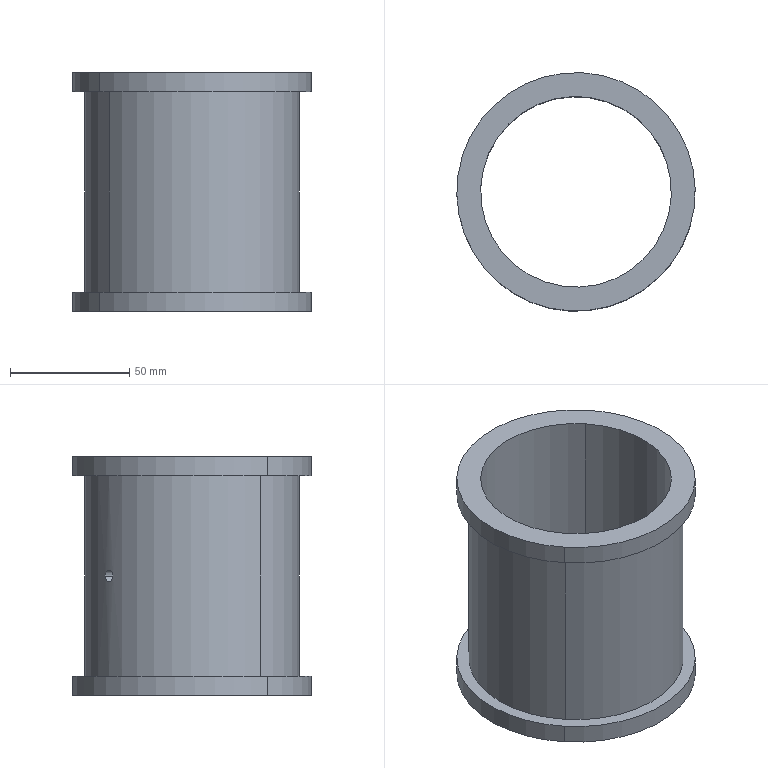Component | SolidWorks | 18Bushing-1 | 1 solid | 14 faces | box 100 x 100 x 100 mm | volume 157296 mm3 | cylinder 10 | plane 4 | commonest cylinder face diameters 100 x4 5 x2 80 x2 90 x2
STEP:
#1=COLOUR_RGB('',0.7922,0.8196,0.9333);
#2=FILL_AREA_STYLE_COLOUR('',#1);
#3=FILL_AREA_STYLE('',(#2));
#4=SURFACE_STYLE_FILL_AREA(#3);
#5=SURFACE_SIDE_STYLE('',(#4));
#6=SURFACE_STYLE_USAGE(.BOTH.,#5);
#7=PRESENTATION_STYLE_ASSIGNMENT((#6));
#8=CARTESIAN_POINT('',(0.5247,7.013,16.299));
#9=VERTEX_POINT('',#8);
#10=CARTESIAN_POINT('',(0.3725,6.888,16.299));
#11=VERTEX_POINT('',#10);
#12=CARTESIAN_POINT('',(0.5247,7.013,16.299));
#13=CARTESIAN_POINT('',(0.5247,7.013,16.306));
#14=CARTESIAN_POINT('',(0.5242,7.013,16.312));
#15=CARTESIAN_POINT('',(0.5221,7.011,16.325));
#16=CARTESIAN_POINT('',(0.5206,7.01,16.331));
#17=CARTESIAN_POINT('',(0.5147,7.006,16.349));
#18=CARTESIAN_POINT('',(0.5088,7.002,16.36));
#19=CARTESIAN_POINT('',(0.4979,6.993,16.373));
#20=CARTESIAN_POINT('',(0.4939,6.99,16.377));
#21=CARTESIAN_POINT('',(0.4854,6.984,16.385));
#22=CARTESIAN_POINT('',(0.481,6.98,16.388));
#23=CARTESIAN_POINT('',(0.4716,6.973,16.393));
#24=CARTESIAN_POINT('',(0.4667,6.969,16.394));
#25=CARTESIAN_POINT('',(0.4569,6.961,16.397));
#26=CARTESIAN_POINT('',(0.4519,6.957,16.398));
#27=CARTESIAN_POINT('',(0.4419,6.949,16.398));
#28=CARTESIAN_POINT('',(0.4369,6.945,16.397));
#29=CARTESIAN_POINT('',(0.4273,6.937,16.395));
#30=CARTESIAN_POINT('',(0.4225,6.933,16.393));
#31=CARTESIAN_POINT('',(0.4135,6.925,16.388));
#32=CARTESIAN_POINT('',(0.4092,6.921,16.385));
#33=CARTESIAN_POINT('',(0.4011,6.914,16.378));
#34=CARTESIAN_POINT('',(0.3973,6.911,16.373));
#35=CARTESIAN_POINT('',(0.3905,6.905,16.364));
#36=CARTESIAN_POINT('',(0.3875,6.902,16.359));
#37=CARTESIAN_POINT('',(0.3821,6.897,16.349));
#38=CARTESIAN_POINT('',(0.3799,6.895,16.343));
#39=CARTESIAN_POINT('',(0.3744,6.89,16.325));
#40=CARTESIAN_POINT('',(0.3725,6.888,16.312));
#41=CARTESIAN_POINT('',(0.3725,6.888,16.299));
#42=B_SPLINE_CURVE_WITH_KNOTS('',3,(#12,#13,#14,#15,#16,#17,#18,#19,#20,#21,#22,#23,#24,#25,#26,#27,#28,#29,#30,#31,#32,#33,#34,#35,#36,#37,#38,#39,#40,#41),.UNSPECIFIED.,.F.,.F.,(4,2,2,2,2,2,2,2,2,2,2,2,2,2,4),(0.007818,0.008306,0.008795,0.009772,0.01026,0.01075,0.01124,0.01173,0.01221,0.0127,0.01319,0.01368,0.01417,0.01466,0.01563),.UNSPECIFIED.);
#43=EDGE_CURVE('',#9,#11,#42,.T.);
#44=ORIENTED_EDGE('',*,*,#43,.F.);
#45=CARTESIAN_POINT('',(0.6497,6.861,16.299));
#46=VERTEX_POINT('',#45);
#47=CARTESIAN_POINT('',(0.3981,7.168,16.299));
#48=DIRECTION('',(0.6341,-0.7732,0.));
#49=VECTOR('',#48,39.37);
#50=LINE('',#47,#49);
#51=EDGE_CURVE('',#9,#46,#50,.T.);
#52=ORIENTED_EDGE('',*,*,#51,.T.);
#53=CARTESIAN_POINT('',(0.4975,6.736,16.299));
#54=VERTEX_POINT('',#53);
#55=CARTESIAN_POINT('',(0.4975,6.736,16.299));
#56=CARTESIAN_POINT('',(0.4975,6.736,16.306));
#57=CARTESIAN_POINT('',(0.498,6.736,16.312));
#58=CARTESIAN_POINT('',(0.4998,6.738,16.325));
#59=CARTESIAN_POINT('',(0.5012,6.739,16.331));
#60=CARTESIAN_POINT('',(0.5048,6.743,16.343));
#61=CARTESIAN_POINT('',(0.5071,6.745,16.349));
#62=CARTESIAN_POINT('',(0.5124,6.75,16.359));
#63=CARTESIAN_POINT('',(0.5155,6.752,16.364));
#64=CARTESIAN_POINT('',(0.5222,6.758,16.373));
#65=CARTESIAN_POINT('',(0.5259,6.762,16.377));
#66=CARTESIAN_POINT('',(0.534,6.769,16.385));
#67=CARTESIAN_POINT('',(0.5383,6.773,16.388));
#68=CARTESIAN_POINT('',(0.5473,6.78,16.393));
#69=CARTESIAN_POINT('',(0.552,6.784,16.394));
#70=CARTESIAN_POINT('',(0.5618,6.793,16.397));
#71=CARTESIAN_POINT('',(0.5667,6.797,16.398));
#72=CARTESIAN_POINT('',(0.5766,6.805,16.398));
#73=CARTESIAN_POINT('',(0.5817,6.809,16.397));
#74=CARTESIAN_POINT('',(0.5915,6.817,16.394));
#75=CARTESIAN_POINT('',(0.5963,6.821,16.393));
#76=CARTESIAN_POINT('',(0.6057,6.828,16.388));
#77=CARTESIAN_POINT('',(0.6103,6.831,16.385));
#78=CARTESIAN_POINT('',(0.6188,6.838,16.377));
#79=CARTESIAN_POINT('',(0.6228,6.841,16.373));
#80=CARTESIAN_POINT('',(0.6301,6.846,16.364));
#81=CARTESIAN_POINT('',(0.6334,6.849,16.359));
#82=CARTESIAN_POINT('',(0.6392,6.853,16.349));
#83=CARTESIAN_POINT('',(0.6416,6.855,16.343));
#84=CARTESIAN_POINT('',(0.6456,6.858,16.331));
#85=CARTESIAN_POINT('',(0.6472,6.859,16.325));
#86=CARTESIAN_POINT('',(0.6492,6.86,16.312));
#87=CARTESIAN_POINT('',(0.6497,6.861,16.306));
#88=CARTESIAN_POINT('',(0.6497,6.861,16.299));
#89=B_SPLINE_CURVE_WITH_KNOTS('',3,(#55,#56,#57,#58,#59,#60,#61,#62,#63,#64,#65,#66,#67,#68,#69,#70,#71,#72,#73,#74,#75,#76,#77,#78,#79,#80,#81,#82,#83,#84,#85,#86,#87,#88),.UNSPECIFIED.,.F.,.F.,(4,2,2,2,2,2,2,2,2,2,2,2,2,2,2,2,4),(0.,0.0004886,0.0009773,0.001466,0.001955,0.002443,0.002932,0.00342,0.003909,0.004398,0.004886,0.005375,0.005864,0.006352,0.006841,0.007329,0.007818),.UNSPECIFIED.);
#90=EDGE_CURVE('',#54,#46,#89,.T.);
#91=ORIENTED_EDGE('',*,*,#90,.F.);
#92=CARTESIAN_POINT('',(0.2459,7.043,16.299));
#93=DIRECTION('',(0.6341,-0.7732,0.));
#94=VECTOR('',#93,39.37);
#95=LINE('',#92,#94);
#96=EDGE_CURVE('',#11,#54,#95,.T.);
#97=ORIENTED_EDGE('',*,*,#96,.F.);
#98=EDGE_LOOP('',(#44,#52,#91,#97));
#99=FACE_OUTER_BOUND('',#98,.T.);
#100=CARTESIAN_POINT('',(0.322,7.105,16.299));
#101=DIRECTION('',(0.6341,-0.7732,0.));
#102=DIRECTION('',(-0.7732,-0.6341,0.));
#103=AXIS2_PLACEMENT_3D('',#100,#101,#102);
#104=CYLINDRICAL_SURFACE('',#103,0.09843);
#105=ADVANCED_FACE('',(#99),#104,.F.);
#106=ORIENTED_EDGE('',*,*,#90,.T.);
#107=CARTESIAN_POINT('',(0.6497,6.861,16.299));
#108=CARTESIAN_POINT('',(0.6497,6.861,16.293));
#109=CARTESIAN_POINT('',(0.6492,6.86,16.286));
#110=CARTESIAN_POINT('',(0.6472,6.859,16.274));
#111=CARTESIAN_POINT('',(0.6456,6.858,16.267));
#112=CARTESIAN_POINT('',(0.6397,6.853,16.25));
#113=CARTESIAN_POINT('',(0.6338,6.849,16.239));
#114=CARTESIAN_POINT('',(0.6229,6.841,16.225));
#115=CARTESIAN_POINT('',(0.6188,6.838,16.221));
#116=CARTESIAN_POINT('',(0.6103,6.831,16.214));
#117=CARTESIAN_POINT('',(0.6058,6.828,16.211));
#118=CARTESIAN_POINT('',(0.5965,6.821,16.206));
#119=CARTESIAN_POINT('',(0.5915,6.817,16.204));
#120=CARTESIAN_POINT('',(0.5817,6.809,16.201));
#121=CARTESIAN_POINT('',(0.5767,6.805,16.201));
#122=CARTESIAN_POINT('',(0.5667,6.797,16.201));
#123=CARTESIAN_POINT('',(0.5618,6.793,16.201));
#124=CARTESIAN_POINT('',(0.5521,6.784,16.204));
#125=CARTESIAN_POINT('',(0.5474,6.78,16.206));
#126=CARTESIAN_POINT('',(0.5383,6.773,16.211));
#127=CARTESIAN_POINT('',(0.5341,6.769,16.214));
#128=CARTESIAN_POINT('',(0.526,6.762,16.221));
#129=CARTESIAN_POINT('',(0.5222,6.758,16.225));
#130=CARTESIAN_POINT('',(0.5155,6.752,16.234));
#131=CARTESIAN_POINT('',(0.5125,6.75,16.239));
#132=CARTESIAN_POINT('',(0.5071,6.745,16.25));
#133=CARTESIAN_POINT('',(0.5049,6.743,16.256));
#134=CARTESIAN_POINT('',(0.4994,6.738,16.273));
#135=CARTESIAN_POINT('',(0.4975,6.736,16.286));
#136=CARTESIAN_POINT('',(0.4975,6.736,16.299));
#137=B_SPLINE_CURVE_WITH_KNOTS('',3,(#107,#108,#109,#110,#111,#112,#113,#114,#115,#116,#117,#118,#119,#120,#121,#122,#123,#124,#125,#126,#127,#128,#129,#130,#131,#132,#133,#134,#135,#136),.UNSPECIFIED.,.F.,.F.,(4,2,2,2,2,2,2,2,2,2,2,2,2,2,4),(0.007818,0.008307,0.008795,0.009772,0.01026,0.01075,0.01124,0.01173,0.01221,0.0127,0.01319,0.01368,0.01417,0.01466,0.01563),.UNSPECIFIED.);
#138=EDGE_CURVE('',#46,#54,#137,.T.);
#139=ORIENTED_EDGE('',*,*,#138,.T.);
#140=EDGE_LOOP('',(#106,#139));
#141=FACE_BOUND('',#140,.T.);
#142=CARTESIAN_POINT('',(0.3526,4.584,18.268));
#143=VERTEX_POINT('',#142);
#144=CARTESIAN_POINT('',(2.788,6.582,18.268));
#145=VERTEX_POINT('',#144);
#146=CARTESIAN_POINT('',(1.57,5.583,18.268));
#147=DIRECTION('',(0.,0.,-1.));
#148=DIRECTION('',(0.7732,0.6341,0.));
#149=AXIS2_PLACEMENT_3D('',#146,#147,#148);
#150=CIRCLE('',#149,1.575);
#151=EDGE_CURVE('',#143,#145,#150,.T.);
#152=ORIENTED_EDGE('',*,*,#151,.F.);
#153=CARTESIAN_POINT('',(0.3526,4.584,14.331));
#154=VERTEX_POINT('',#153);
#155=CARTESIAN_POINT('',(0.3526,4.584,18.268));
#156=DIRECTION('',(0.,0.,-1.));
#157=VECTOR('',#156,39.37);
#158=LINE('',#155,#157);
#159=EDGE_CURVE('',#143,#154,#158,.T.);
#160=ORIENTED_EDGE('',*,*,#159,.T.);
#161=CARTESIAN_POINT('',(2.788,6.582,14.331));
#162=VERTEX_POINT('',#161);
#163=CARTESIAN_POINT('',(1.57,5.583,14.331));
#164=DIRECTION('',(0.,0.,-1.));
#165=DIRECTION('',(0.7732,0.6341,0.));
#166=AXIS2_PLACEMENT_3D('',#163,#164,#165);
#167=CIRCLE('',#166,1.575);
#168=EDGE_CURVE('',#154,#162,#167,.T.);
#169=ORIENTED_EDGE('',*,*,#168,.T.);
#170=CARTESIAN_POINT('',(2.788,6.582,18.268));
#171=DIRECTION('',(0.,0.,-1.));
#172=VECTOR('',#171,39.37);
#173=LINE('',#170,#172);
#174=EDGE_CURVE('',#145,#162,#173,.T.);
#175=ORIENTED_EDGE('',*,*,#174,.F.);
#176=EDGE_LOOP('',(#152,#160,#169,#175));
#177=FACE_OUTER_BOUND('',#176,.T.);
#178=CARTESIAN_POINT('',(1.57,5.583,18.268));
#179=DIRECTION('',(0.,0.,-1.));
#180=DIRECTION('',(0.7732,0.6341,0.));
#181=AXIS2_PLACEMENT_3D('',#178,#179,#180);
#182=CYLINDRICAL_SURFACE('',#181,1.575);
#183=ADVANCED_FACE('',(#141,#177),#182,.F.);
#184=CARTESIAN_POINT('',(3.092,6.831,14.331));
#185=VERTEX_POINT('',#184);
#186=CARTESIAN_POINT('',(0.04813,4.335,14.331));
#187=VERTEX_POINT('',#186);
#188=CARTESIAN_POINT('',(1.57,5.583,14.331));
#189=DIRECTION('',(0.,0.,-1.));
#190=DIRECTION('',(0.7732,0.6341,0.));
#191=AXIS2_PLACEMENT_3D('',#188,#189,#190);
#192=CIRCLE('',#191,1.969);
#193=EDGE_CURVE('',#185,#187,#192,.T.);
#194=ORIENTED_EDGE('',*,*,#193,.F.);
#195=CARTESIAN_POINT('',(3.092,6.831,14.646));
#196=VERTEX_POINT('',#195);
#197=CARTESIAN_POINT('',(3.092,6.831,14.331));
#198=DIRECTION('',(0.,0.,1.));
#199=VECTOR('',#198,39.37);
#200=LINE('',#197,#199);
#201=EDGE_CURVE('',#185,#196,#200,.T.);
#202=ORIENTED_EDGE('',*,*,#201,.T.);
#203=CARTESIAN_POINT('',(0.04813,4.335,14.646));
#204=VERTEX_POINT('',#203);
#205=CARTESIAN_POINT('',(1.57,5.583,14.646));
#206=DIRECTION('',(0.,0.,-1.));
#207=DIRECTION('',(0.7732,0.6341,0.));
#208=AXIS2_PLACEMENT_3D('',#205,#206,#207);
#209=CIRCLE('',#208,1.969);
#210=EDGE_CURVE('',#196,#204,#209,.T.);
#211=ORIENTED_EDGE('',*,*,#210,.T.);
#212=CARTESIAN_POINT('',(0.04813,4.335,14.331));
#213=DIRECTION('',(0.,0.,1.));
#214=VECTOR('',#213,39.37);
#215=LINE('',#212,#214);
#216=EDGE_CURVE('',#187,#204,#215,.T.);
#217=ORIENTED_EDGE('',*,*,#216,.F.);
#218=EDGE_LOOP('',(#194,#202,#211,#217));
#219=FACE_OUTER_BOUND('',#218,.T.);
#220=CARTESIAN_POINT('',(1.57,5.583,14.331));
#221=DIRECTION('',(0.,0.,1.));
#222=DIRECTION('',(-0.7732,-0.6341,0.));
#223=AXIS2_PLACEMENT_3D('',#220,#221,#222);
#224=CYLINDRICAL_SURFACE('',#223,1.969);
#225=ADVANCED_FACE('',(#219),#224,.T.);
#226=CARTESIAN_POINT('',(2.94,6.706,14.646));
#227=VERTEX_POINT('',#226);
#228=CARTESIAN_POINT('',(0.2003,4.46,14.646));
#229=VERTEX_POINT('',#228);
#230=CARTESIAN_POINT('',(1.57,5.583,14.646));
#231=DIRECTION('',(0.,0.,-1.));
#232=DIRECTION('',(0.7732,0.6341,0.));
#233=AXIS2_PLACEMENT_3D('',#230,#231,#232);
#234=CIRCLE('',#233,1.772);
#235=EDGE_CURVE('',#227,#229,#234,.T.);
#236=ORIENTED_EDGE('',*,*,#235,.F.);
#237=CARTESIAN_POINT('',(2.94,6.706,17.953));
#238=VERTEX_POINT('',#237);
#239=CARTESIAN_POINT('',(2.94,6.706,14.646));
#240=DIRECTION('',(0.,0.,1.));
#241=VECTOR('',#240,39.37);
#242=LINE('',#239,#241);
#243=EDGE_CURVE('',#227,#238,#242,.T.);
#244=ORIENTED_EDGE('',*,*,#243,.T.);
#245=CARTESIAN_POINT('',(0.2003,4.46,17.953));
#246=VERTEX_POINT('',#245);
#247=CARTESIAN_POINT('',(1.57,5.583,17.953));
#248=DIRECTION('',(0.,0.,-1.));
#249=DIRECTION('',(0.7732,0.6341,0.));
#250=AXIS2_PLACEMENT_3D('',#247,#248,#249);
#251=CIRCLE('',#250,1.772);
#252=EDGE_CURVE('',#238,#246,#251,.T.);
#253=ORIENTED_EDGE('',*,*,#252,.T.);
#254=CARTESIAN_POINT('',(0.2003,4.46,14.646));
#255=DIRECTION('',(0.,0.,1.));
#256=VECTOR('',#255,39.37);
#257=LINE('',#254,#256);
#258=EDGE_CURVE('',#229,#246,#257,.T.);
#259=ORIENTED_EDGE('',*,*,#258,.F.);
#260=EDGE_LOOP('',(#236,#244,#253,#259));
#261=FACE_OUTER_BOUND('',#260,.T.);
#262=CARTESIAN_POINT('',(1.57,5.583,14.646));
#263=DIRECTION('',(0.,0.,1.));
#264=DIRECTION('',(-0.7732,-0.6341,0.));
#265=AXIS2_PLACEMENT_3D('',#262,#263,#264);
#266=CYLINDRICAL_SURFACE('',#265,1.772);
#267=ADVANCED_FACE('',(#261),#266,.T.);
#268=CARTESIAN_POINT('',(3.092,6.831,17.953));
#269=VERTEX_POINT('',#268);
#270=CARTESIAN_POINT('',(0.04813,4.335,17.953));
#271=VERTEX_POINT('',#270);
#272=CARTESIAN_POINT('',(1.57,5.583,17.953));
#273=DIRECTION('',(0.,0.,-1.));
#274=DIRECTION('',(0.7732,0.6341,0.));
#275=AXIS2_PLACEMENT_3D('',#272,#273,#274);
#276=CIRCLE('',#275,1.969);
#277=EDGE_CURVE('',#269,#271,#276,.T.);
#278=ORIENTED_EDGE('',*,*,#277,.F.);
#279=CARTESIAN_POINT('',(3.092,6.831,18.268));
#280=VERTEX_POINT('',#279);
#281=CARTESIAN_POINT('',(3.092,6.831,17.953));
#282=DIRECTION('',(0.,0.,1.));
#283=VECTOR('',#282,39.37);
#284=LINE('',#281,#283);
#285=EDGE_CURVE('',#269,#280,#284,.T.);
#286=ORIENTED_EDGE('',*,*,#285,.T.);
#287=CARTESIAN_POINT('',(0.04813,4.335,18.268));
#288=VERTEX_POINT('',#287);
#289=CARTESIAN_POINT('',(1.57,5.583,18.268));
#290=DIRECTION('',(0.,0.,-1.));
#291=DIRECTION('',(0.7732,0.6341,0.));
#292=AXIS2_PLACEMENT_3D('',#289,#290,#291);
#293=CIRCLE('',#292,1.969);
#294=EDGE_CURVE('',#280,#288,#293,.T.);
#295=ORIENTED_EDGE('',*,*,#294,.T.);
#296=CARTESIAN_POINT('',(0.04813,4.335,17.953));
#297=DIRECTION('',(0.,0.,1.));
#298=VECTOR('',#297,39.37);
#299=LINE('',#296,#298);
#300=EDGE_CURVE('',#271,#288,#299,.T.);
#301=ORIENTED_EDGE('',*,*,#300,.F.);
#302=EDGE_LOOP('',(#278,#286,#295,#301));
#303=FACE_OUTER_BOUND('',#302,.T.);
#304=CARTESIAN_POINT('',(1.57,5.583,17.953));
#305=DIRECTION('',(0.,0.,1.));
#306=DIRECTION('',(-0.7732,-0.6341,0.));
#307=AXIS2_PLACEMENT_3D('',#304,#305,#306);
#308=CYLINDRICAL_SURFACE('',#307,1.969);
#309=ADVANCED_FACE('',(#303),#308,.T.);
#310=ORIENTED_EDGE('',*,*,#285,.F.);
#311=CARTESIAN_POINT('',(1.57,5.583,17.953));
#312=DIRECTION('',(0.,0.,-1.));
#313=DIRECTION('',(0.7732,0.6341,0.));
#314=AXIS2_PLACEMENT_3D('',#311,#312,#313);
#315=CIRCLE('',#314,1.969);
#316=EDGE_CURVE('',#271,#269,#315,.T.);
#317=ORIENTED_EDGE('',*,*,#316,.F.);
#318=ORIENTED_EDGE('',*,*,#300,.T.);
#319=CARTESIAN_POINT('',(1.57,5.583,18.268));
#320=DIRECTION('',(0.,0.,-1.));
#321=DIRECTION('',(0.7732,0.6341,0.));
#322=AXIS2_PLACEMENT_3D('',#319,#320,#321);
#323=CIRCLE('',#322,1.969);
#324=EDGE_CURVE('',#288,#280,#323,.T.);
#325=ORIENTED_EDGE('',*,*,#324,.T.);
#326=EDGE_LOOP('',(#310,#317,#318,#325));
#327=FACE_OUTER_BOUND('',#326,.T.);
#328=CARTESIAN_POINT('',(1.57,5.583,17.953));
#329=DIRECTION('',(0.,0.,1.));
#330=DIRECTION('',(-0.7732,-0.6341,0.));
#331=AXIS2_PLACEMENT_3D('',#328,#329,#330);
#332=CYLINDRICAL_SURFACE('',#331,1.969);
#333=ADVANCED_FACE('',(#327),#332,.T.);
#334=CARTESIAN_POINT('',(1.57,5.583,17.953));
#335=DIRECTION('',(0.,0.,-1.));
#336=DIRECTION('',(0.7732,0.6341,0.));
#337=AXIS2_PLACEMENT_3D('',#334,#335,#336);
#338=CIRCLE('',#337,1.772);
#339=EDGE_CURVE('',#246,#238,#338,.T.);
#340=ORIENTED_EDGE('',*,*,#339,.F.);
#341=ORIENTED_EDGE('',*,*,#252,.F.);
#342=EDGE_LOOP('',(#340,#341));
#343=FACE_BOUND('',#342,.T.);
#344=ORIENTED_EDGE('',*,*,#316,.T.);
#345=ORIENTED_EDGE('',*,*,#277,.T.);
#346=EDGE_LOOP('',(#344,#345));
#347=FACE_OUTER_BOUND('',#346,.T.);
#348=CARTESIAN_POINT('',(1.57,5.583,17.953));
#349=DIRECTION('',(0.,0.,-1.));
#350=DIRECTION('',(0.7732,0.6341,0.));
#351=AXIS2_PLACEMENT_3D('',#348,#349,#350);
#352=PLANE('',#351);
#353=ADVANCED_FACE('',(#343,#347),#352,.T.);
#354=CARTESIAN_POINT('',(1.57,5.583,18.268));
#355=DIRECTION('',(0.,0.,-1.));
#356=DIRECTION('',(0.7732,0.6341,0.));
#357=AXIS2_PLACEMENT_3D('',#354,#355,#356);
#358=CIRCLE('',#357,1.575);
#359=EDGE_CURVE('',#145,#143,#358,.T.);
#360=ORIENTED_EDGE('',*,*,#359,.T.);
#361=ORIENTED_EDGE('',*,*,#151,.T.);
#362=EDGE_LOOP('',(#360,#361));
#363=FACE_BOUND('',#362,.T.);
#364=ORIENTED_EDGE('',*,*,#324,.F.);
#365=ORIENTED_EDGE('',*,*,#294,.F.);
#366=EDGE_LOOP('',(#364,#365));
#367=FACE_OUTER_BOUND('',#366,.T.);
#368=CARTESIAN_POINT('',(1.57,5.583,18.268));
#369=DIRECTION('',(0.,0.,-1.));
#370=DIRECTION('',(0.7732,0.6341,0.));
#371=AXIS2_PLACEMENT_3D('',#368,#369,#370);
#372=PLANE('',#371);
#373=ADVANCED_FACE('',(#363,#367),#372,.F.);
#374=ORIENTED_EDGE('',*,*,#243,.F.);
#375=CARTESIAN_POINT('',(1.57,5.583,14.646));
#376=DIRECTION('',(0.,0.,-1.));
#377=DIRECTION('',(0.7732,0.6341,0.));
#378=AXIS2_PLACEMENT_3D('',#375,#376,#377);
#379=CIRCLE('',#378,1.772);
#380=EDGE_CURVE('',#229,#227,#379,.T.);
#381=ORIENTED_EDGE('',*,*,#380,.F.);
#382=ORIENTED_EDGE('',*,*,#258,.T.);
#383=ORIENTED_EDGE('',*,*,#339,.T.);
#384=EDGE_LOOP('',(#374,#381,#382,#383));
#385=FACE_OUTER_BOUND('',#384,.T.);
#386=CARTESIAN_POINT('',(0.3725,6.888,16.299));
#387=CARTESIAN_POINT('',(0.3725,6.888,16.293));
#388=CARTESIAN_POINT('',(0.3729,6.889,16.286));
#389=CARTESIAN_POINT('',(0.3748,6.891,16.274));
#390=CARTESIAN_POINT('',(0.3762,6.892,16.267));
#391=CARTESIAN_POINT('',(0.3798,6.895,16.256));
#392=CARTESIAN_POINT('',(0.3821,6.897,16.25));
#393=CARTESIAN_POINT('',(0.3874,6.902,16.239));
#394=CARTESIAN_POINT('',(0.3905,6.905,16.234));
#395=CARTESIAN_POINT('',(0.3973,6.911,16.225));
#396=CARTESIAN_POINT('',(0.401,6.914,16.221));
#397=CARTESIAN_POINT('',(0.4091,6.921,16.214));
#398=CARTESIAN_POINT('',(0.4135,6.925,16.211));
#399=CARTESIAN_POINT('',(0.4225,6.933,16.206));
#400=CARTESIAN_POINT('',(0.4272,6.937,16.204));
#401=CARTESIAN_POINT('',(0.4369,6.945,16.201));
#402=CARTESIAN_POINT('',(0.4418,6.949,16.201));
#403=CARTESIAN_POINT('',(0.4518,6.957,16.201));
#404=CARTESIAN_POINT('',(0.4568,6.961,16.201));
#405=CARTESIAN_POINT('',(0.4667,6.969,16.204));
#406=CARTESIAN_POINT('',(0.4715,6.973,16.206));
#407=CARTESIAN_POINT('',(0.4809,6.98,16.211));
#408=CARTESIAN_POINT('',(0.4854,6.984,16.214));
#409=CARTESIAN_POINT('',(0.4939,6.99,16.221));
#410=CARTESIAN_POINT('',(0.4978,6.993,16.225));
#411=CARTESIAN_POINT('',(0.5052,6.999,16.234));
#412=CARTESIAN_POINT('',(0.5084,7.001,16.239));
#413=CARTESIAN_POINT('',(0.5142,7.006,16.25));
#414=CARTESIAN_POINT('',(0.5166,7.007,16.256));
#415=CARTESIAN_POINT('',(0.5206,7.01,16.268));
#416=CARTESIAN_POINT('',(0.5221,7.011,16.274));
#417=CARTESIAN_POINT('',(0.5242,7.013,16.286));
#418=CARTESIAN_POINT('',(0.5247,7.013,16.293));
#419=CARTESIAN_POINT('',(0.5247,7.013,16.299));
#420=B_SPLINE_CURVE_WITH_KNOTS('',3,(#386,#387,#388,#389,#390,#391,#392,#393,#394,#395,#396,#397,#398,#399,#400,#401,#402,#403,#404,#405,#406,#407,#408,#409,#410,#411,#412,#413,#414,#415,#416,#417,#418,#419),.UNSPECIFIED.,.F.,.F.,(4,2,2,2,2,2,2,2,2,2,2,2,2,2,2,2,4),(0.,0.0004886,0.0009772,0.001466,0.001954,0.002443,0.002932,0.00342,0.003909,0.004397,0.004886,0.005375,0.005863,0.006352,0.00684,0.007329,0.007818),.UNSPECIFIED.);
#421=EDGE_CURVE('',#11,#9,#420,.T.);
#422=ORIENTED_EDGE('',*,*,#421,.T.);
#423=ORIENTED_EDGE('',*,*,#43,.T.);
#424=EDGE_LOOP('',(#422,#423));
#425=FACE_BOUND('',#424,.T.);
#426=CARTESIAN_POINT('',(1.57,5.583,14.646));
#427=DIRECTION('',(0.,0.,1.));
#428=DIRECTION('',(-0.7732,-0.6341,0.));
#429=AXIS2_PLACEMENT_3D('',#426,#427,#428);
#430=CYLINDRICAL_SURFACE('',#429,1.772);
#431=ADVANCED_FACE('',(#385,#425),#430,.T.);
#432=ORIENTED_EDGE('',*,*,#201,.F.);
#433=CARTESIAN_POINT('',(1.57,5.583,14.331));
#434=DIRECTION('',(0.,0.,-1.));
#435=DIRECTION('',(0.7732,0.6341,0.));
#436=AXIS2_PLACEMENT_3D('',#433,#434,#435);
#437=CIRCLE('',#436,1.969);
#438=EDGE_CURVE('',#187,#185,#437,.T.);
#439=ORIENTED_EDGE('',*,*,#438,.F.);
#440=ORIENTED_EDGE('',*,*,#216,.T.);
#441=CARTESIAN_POINT('',(1.57,5.583,14.646));
#442=DIRECTION('',(0.,0.,-1.));
#443=DIRECTION('',(0.7732,0.6341,0.));
#444=AXIS2_PLACEMENT_3D('',#441,#442,#443);
#445=CIRCLE('',#444,1.969);
#446=EDGE_CURVE('',#204,#196,#445,.T.);
#447=ORIENTED_EDGE('',*,*,#446,.T.);
#448=EDGE_LOOP('',(#432,#439,#440,#447));
#449=FACE_OUTER_BOUND('',#448,.T.);
#450=CARTESIAN_POINT('',(1.57,5.583,14.331));
#451=DIRECTION('',(0.,0.,1.));
#452=DIRECTION('',(-0.7732,-0.6341,0.));
#453=AXIS2_PLACEMENT_3D('',#450,#451,#452);
#454=CYLINDRICAL_SURFACE('',#453,1.969);
#455=ADVANCED_FACE('',(#449),#454,.T.);
#456=CARTESIAN_POINT('',(1.57,5.583,14.331));
#457=DIRECTION('',(0.,0.,-1.));
#458=DIRECTION('',(0.7732,0.6341,0.));
#459=AXIS2_PLACEMENT_3D('',#456,#457,#458);
#460=CIRCLE('',#459,1.575);
#461=EDGE_CURVE('',#162,#154,#460,.T.);
#462=ORIENTED_EDGE('',*,*,#461,.F.);
#463=ORIENTED_EDGE('',*,*,#168,.F.);
#464=EDGE_LOOP('',(#462,#463));
#465=FACE_BOUND('',#464,.T.);
#466=ORIENTED_EDGE('',*,*,#438,.T.);
#467=ORIENTED_EDGE('',*,*,#193,.T.);
#468=EDGE_LOOP('',(#466,#467));
#469=FACE_OUTER_BOUND('',#468,.T.);
#470=CARTESIAN_POINT('',(1.57,5.583,14.331));
#471=DIRECTION('',(0.,0.,-1.));
#472=DIRECTION('',(0.7732,0.6341,0.));
#473=AXIS2_PLACEMENT_3D('',#470,#471,#472);
#474=PLANE('',#473);
#475=ADVANCED_FACE('',(#465,#469),#474,.T.);
#476=ORIENTED_EDGE('',*,*,#380,.T.);
#477=ORIENTED_EDGE('',*,*,#235,.T.);
#478=EDGE_LOOP('',(#476,#477));
#479=FACE_BOUND('',#478,.T.);
#480=ORIENTED_EDGE('',*,*,#446,.F.);
#481=ORIENTED_EDGE('',*,*,#210,.F.);
#482=EDGE_LOOP('',(#480,#481));
#483=FACE_OUTER_BOUND('',#482,.T.);
#484=CARTESIAN_POINT('',(1.57,5.583,14.646));
#485=DIRECTION('',(0.,0.,-1.));
#486=DIRECTION('',(0.7732,0.6341,0.));
#487=AXIS2_PLACEMENT_3D('',#484,#485,#486);
#488=PLANE('',#487);
#489=ADVANCED_FACE('',(#479,#483),#488,.F.);
#490=ORIENTED_EDGE('',*,*,#159,.F.);
#491=ORIENTED_EDGE('',*,*,#359,.F.);
#492=ORIENTED_EDGE('',*,*,#174,.T.);
#493=ORIENTED_EDGE('',*,*,#461,.T.);
#494=EDGE_LOOP('',(#490,#491,#492,#493));
#495=FACE_OUTER_BOUND('',#494,.T.);
#496=CARTESIAN_POINT('',(1.57,5.583,18.268));
#497=DIRECTION('',(0.,0.,-1.));
#498=DIRECTION('',(0.7732,0.6341,0.));
#499=AXIS2_PLACEMENT_3D('',#496,#497,#498);
#500=CYLINDRICAL_SURFACE('',#499,1.575);
#501=ADVANCED_FACE('',(#495),#500,.F.);
#502=ORIENTED_EDGE('',*,*,#51,.F.);
#503=ORIENTED_EDGE('',*,*,#421,.F.);
#504=ORIENTED_EDGE('',*,*,#96,.T.);
#505=ORIENTED_EDGE('',*,*,#138,.F.);
#506=EDGE_LOOP('',(#502,#503,#504,#505));
#507=FACE_OUTER_BOUND('',#506,.T.);
#508=CARTESIAN_POINT('',(0.322,7.105,16.299));
#509=DIRECTION('',(0.6341,-0.7732,0.));
#510=DIRECTION('',(-0.7732,-0.6341,0.));
#511=AXIS2_PLACEMENT_3D('',#508,#509,#510);
#512=CYLINDRICAL_SURFACE('',#511,0.09843);
#513=ADVANCED_FACE('',(#507),#512,.F.);
#514=CLOSED_SHELL('',(#105,#183,#225,#267,#309,#333,#353,#373,#431,#455,#475,#489,#501,#513));
#515=MANIFOLD_SOLID_BREP('',#514);
#516=STYLED_ITEM('',(#7),#515);
#517=PRESENTATION_LAYER_ASSIGNMENT('','',(#516));
#518=(LENGTH_UNIT()NAMED_UNIT(*)SI_UNIT($,.METRE.));
#519=LENGTH_MEASURE_WITH_UNIT(LENGTH_MEASURE(0.0254),#518);
#520=DIMENSIONAL_EXPONENTS(1.,0.,0.,0.,0.,0.,0.);
#521=(CONVERSION_BASED_UNIT('',#519)LENGTH_UNIT()NAMED_UNIT(#520));
#522=UNCERTAINTY_MEASURE_WITH_UNIT(LENGTH_MEASURE(0.00001),#521,'','');
#523=(NAMED_UNIT(*)PLANE_ANGLE_UNIT()SI_UNIT($,.RADIAN.));
#524=(NAMED_UNIT(*)SI_UNIT($,.STERADIAN.)SOLID_ANGLE_UNIT());
#525=(GEOMETRIC_REPRESENTATION_CONTEXT(3)GLOBAL_UNCERTAINTY_ASSIGNED_CONTEXT((#522))GLOBAL_UNIT_ASSIGNED_CONTEXT((#521,#523,#524))REPRESENTATION_CONTEXT('',''));
#526=MECHANICAL_DESIGN_GEOMETRIC_PRESENTATION_REPRESENTATION('',(#516),#525);
#527=CARTESIAN_POINT('',(0.,0.,0.));
#528=DIRECTION('',(0.,0.,1.));
#529=DIRECTION('',(1.,0.,0.));
#530=AXIS2_PLACEMENT_3D('',#527,#528,#529);
#531=(LENGTH_UNIT()NAMED_UNIT(*)SI_UNIT($,.METRE.));
#532=LENGTH_MEASURE_WITH_UNIT(LENGTH_MEASURE(0.0254),#531);
#533=DIMENSIONAL_EXPONENTS(1.,0.,0.,0.,0.,0.,0.);
#534=(CONVERSION_BASED_UNIT('',#532)LENGTH_UNIT()NAMED_UNIT(#533));
#535=UNCERTAINTY_MEASURE_WITH_UNIT(LENGTH_MEASURE(0.00001),#534,'','');
#536=(NAMED_UNIT(*)PLANE_ANGLE_UNIT()SI_UNIT($,.RADIAN.));
#537=(NAMED_UNIT(*)SI_UNIT($,.STERADIAN.)SOLID_ANGLE_UNIT());
#538=(GEOMETRIC_REPRESENTATION_CONTEXT(3)GLOBAL_UNCERTAINTY_ASSIGNED_CONTEXT((#535))GLOBAL_UNIT_ASSIGNED_CONTEXT((#534,#536,#537))REPRESENTATION_CONTEXT('',''));
#539=ADVANCED_BREP_SHAPE_REPRESENTATION('',(#515,#530),#538);